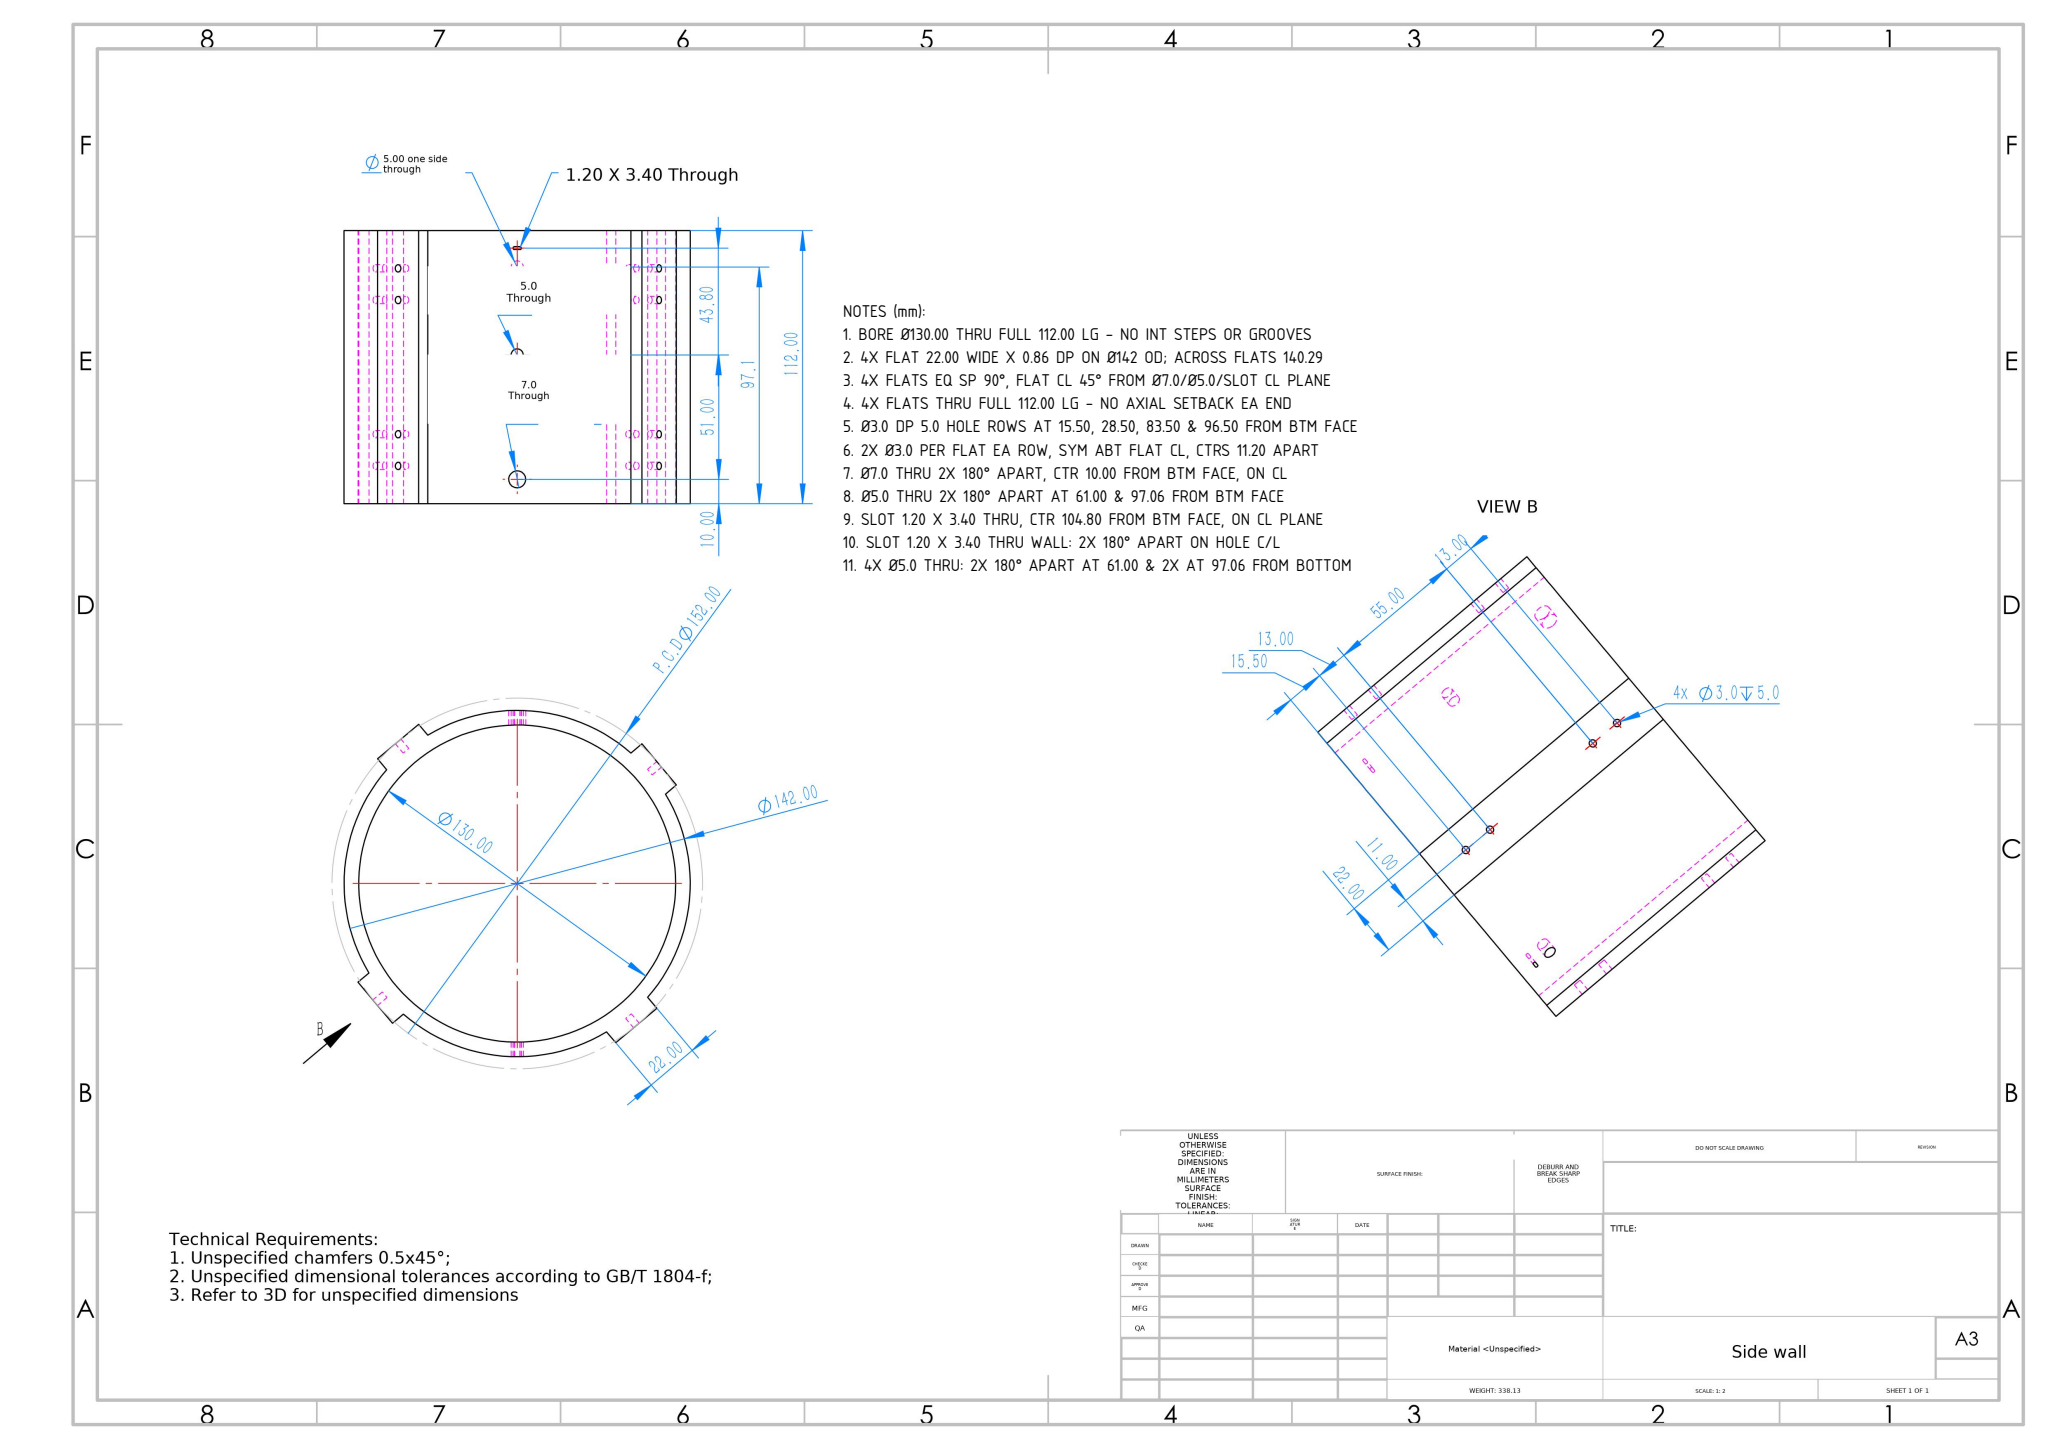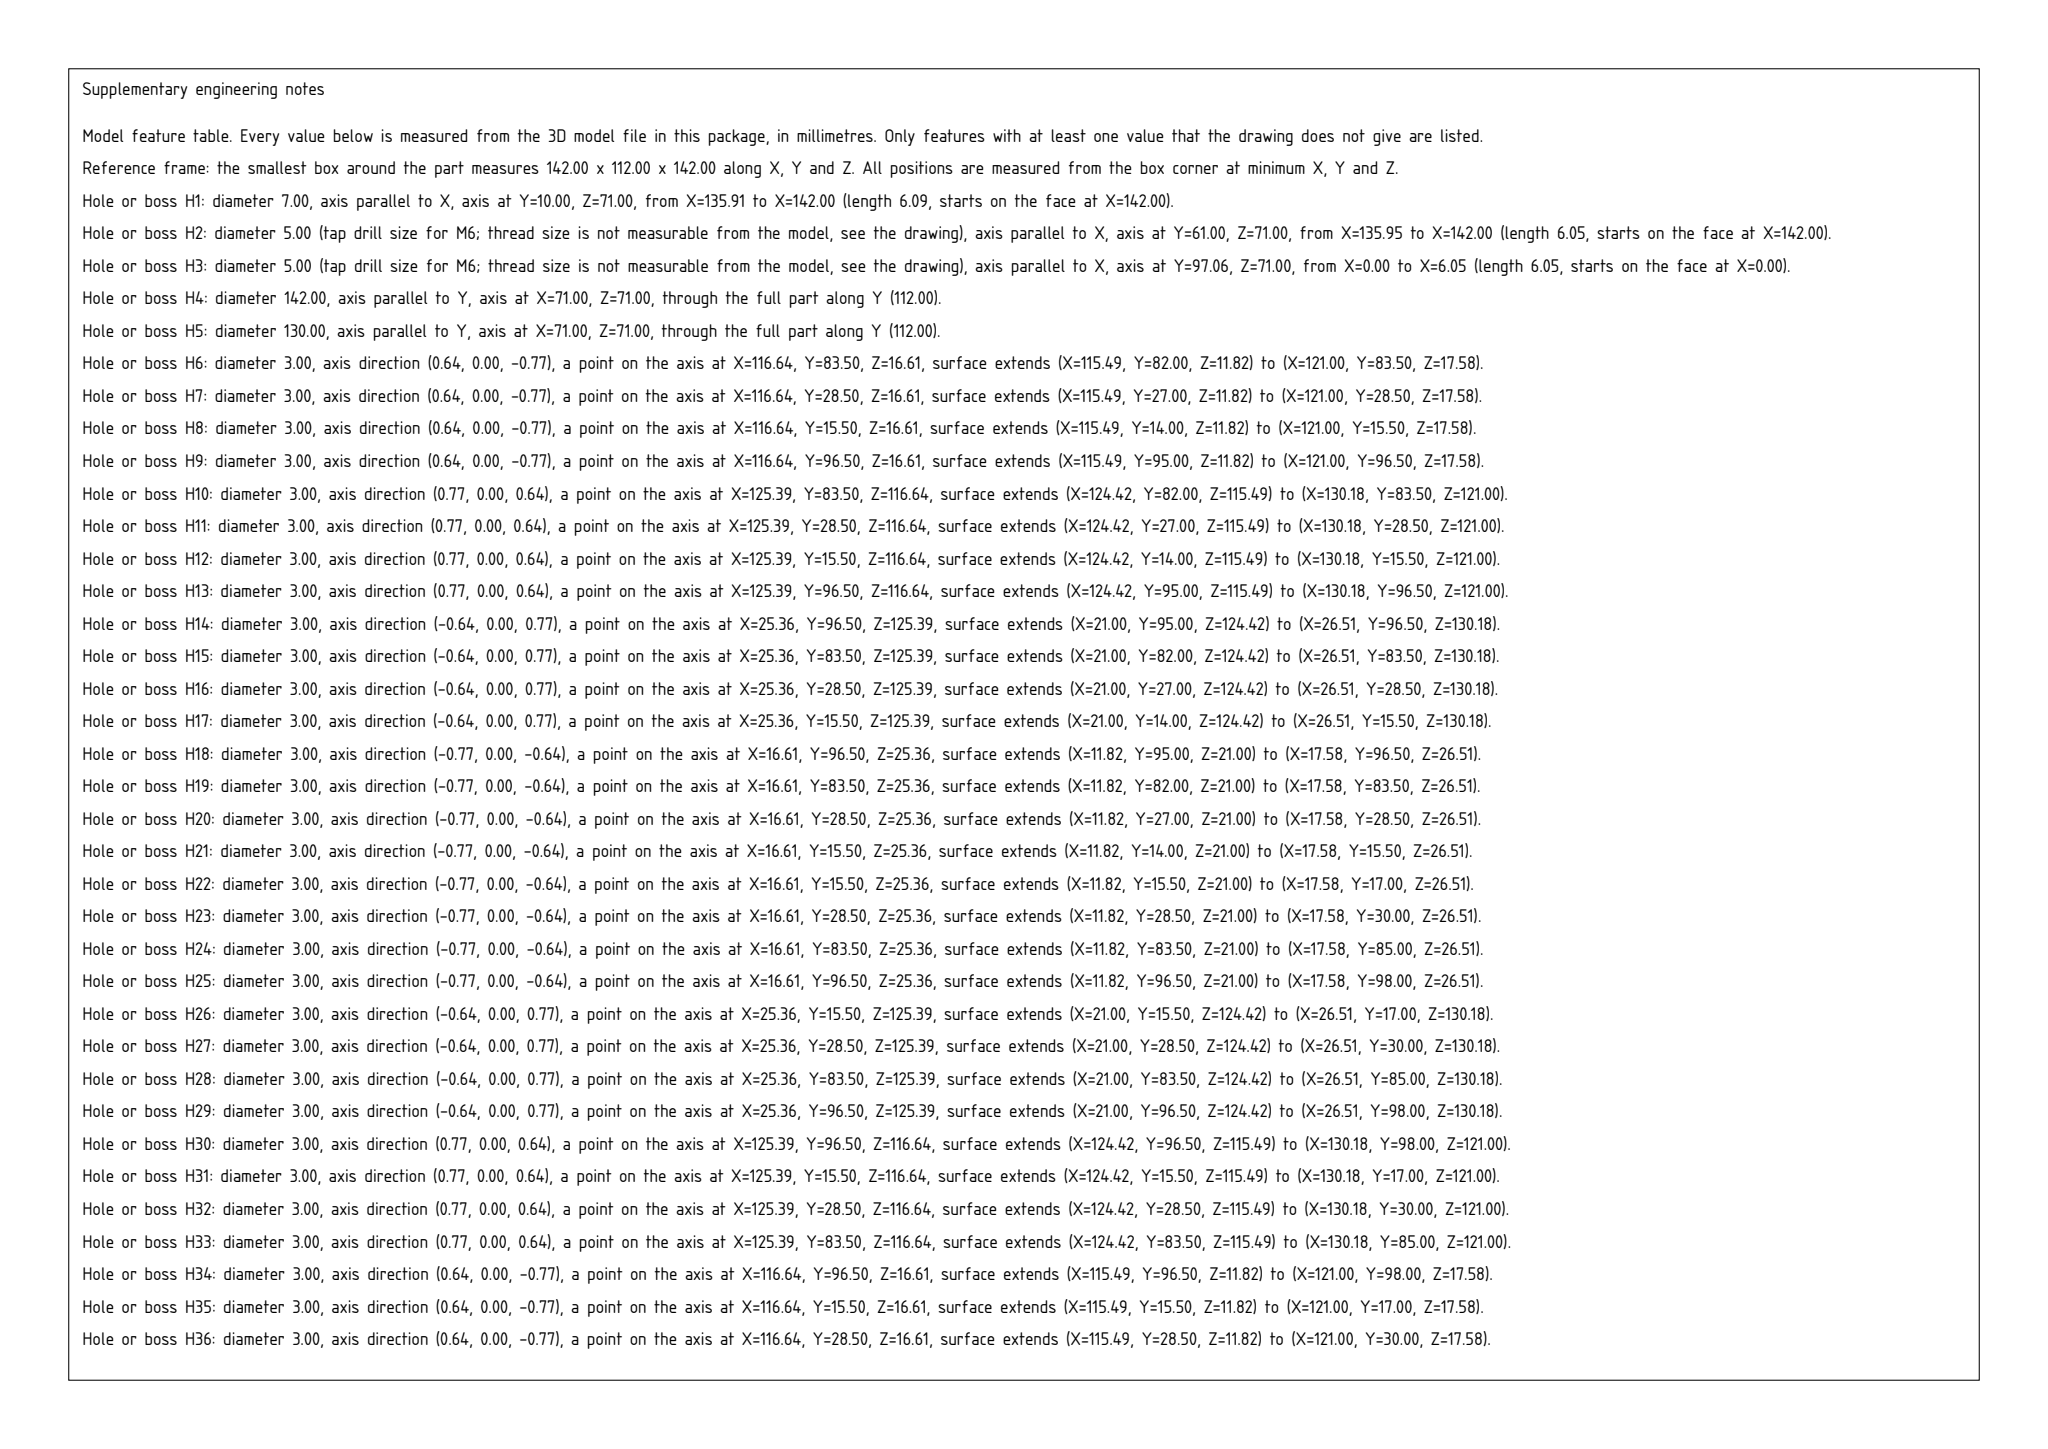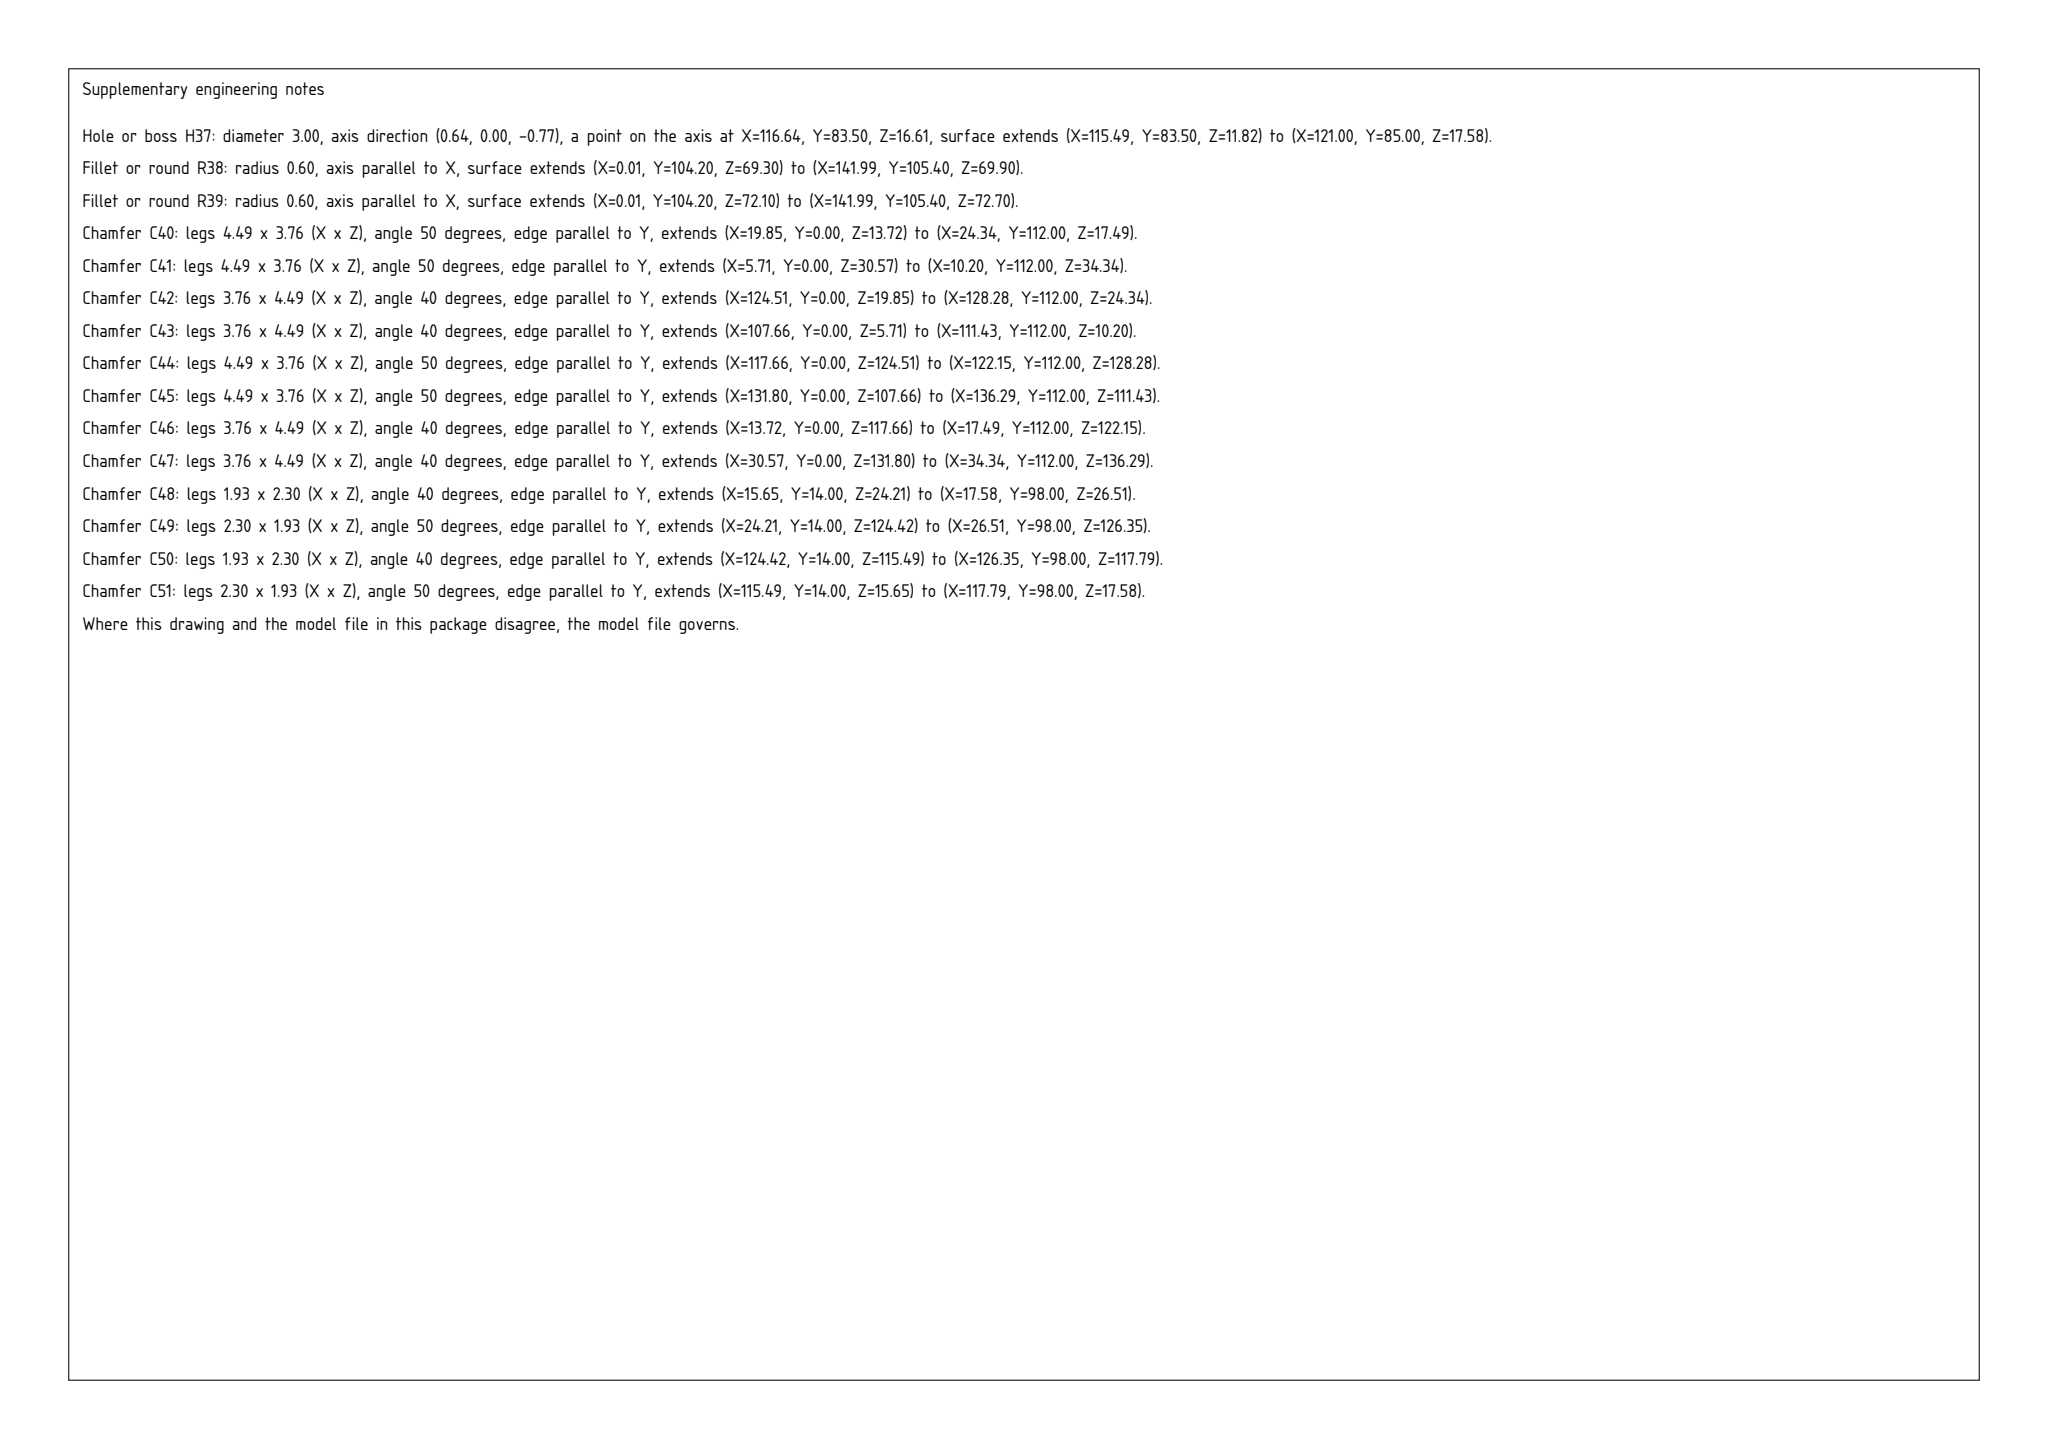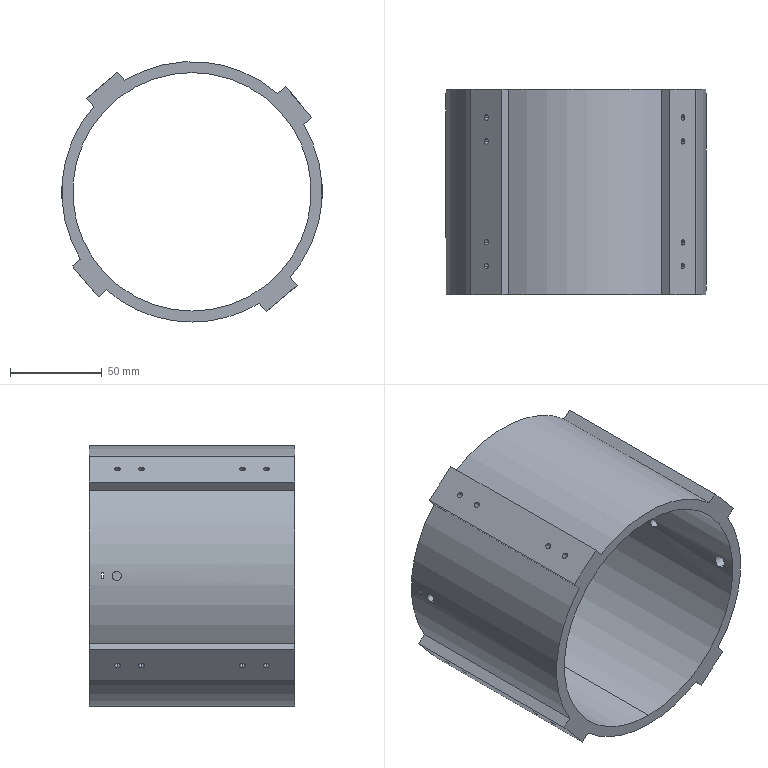Part | SolidWorks | mm | 1 solid | 85 faces | box 142 x 112 x 142 mm | volume 338129 mm3 | cylinder 51 | plane 34 | commonest cylinder face diameters 3 x32 1.2 x6 142 x5 5 x4 7 x2 130 x2
Drawing notes:
BORE Ø130.00 THRU FULL 112.00 LG - NO INT STEPS OR GROOVES | from the solid: Only cyls Ø130 and Ø142, axis y, length 112 full; no other bore faces
4X FLAT 22.00 WIDE X 0.86 DP ON Ø142 OD; ACROSS FLATS 140.29 | from the solid: Ø142 OD split into 5 cyl faces by 4 flats; chord 22 on R71 -> dp 0.857, A/F 140.285
4X FLATS EQ SP 90°, FLAT CL 45° FROM Ø7.0/Ø5.0/SLOT CL PLANE | from the solid: Ø7.0, Ø5.0 & 1.2x3.4 slot on z=71 CL; flat hole pairs centred on the 4 diagonals
4X FLATS THRU FULL 112.00 LG - NO AXIAL SETBACK EA END | from the solid: Ø142 cyl faces each 112.00 long (count 5), bbox y=112.0; flats run end face to end face
Ø3.0 DP 5.0 HOLE ROWS AT 15.50, 28.50, 83.50 & 96.50 FROM BTM FACE | from the solid: Ø3.0 x 5.76 deep cyls at y=15.5, 28.5, 83.5, 96.5 (5.0 flat DP), part 112 lg
2X Ø3.0 PER FLAT EA ROW, SYM ABT FLAT CL, CTRS 11.20 APART | from the solid: Ø3.0 axes at x/z=25.36 & 116.64; pair ctr dist sqrt(7.92²+7.92²)=11.20 on each flat
Ø7.0 THRU 2X 180° APART, CTR 10.00 FROM BTM FACE, ON CL | from the solid: [7.0,'x',[null,10.0,71.0],6.09,2] - z=71 = part CL, y=10 from min face
Ø5.0 THRU 2X 180° APART AT 61.00 & 97.06 FROM BTM FACE | from the solid: [5.0,'x',[null,61.0,71.0],6.05,2] and [5.0,'x',[null,97.06,71.0],6.05,2]
SLOT 1.20 X 3.40 THRU, CTR 104.80 FROM BTM FACE, ON CL PLANE | from the solid: Ø1.2 cyls, axis x, y=104.8, z=69.9 & 72.1 (3.4 overall); planes y=104.2/105.4
SLOT 1.20 X 3.40 THRU WALL: 2X 180° APART ON HOLE C/L | from the solid: dia-1.2 slot-end cyls at y=104.8, z=69.9 & 72.1, axis X, len 6.01 (=wall thk); only 2 wall crossings exist on that X line (x=0-6.01 and 135.99-142), i.e. 2 slots 180° apart on z=71 c/l
4X Ø5.0 THRU: 2X 180° APART AT 61.00 & 2X AT 97.06 FROM BOTTOM | from the solid: dia-5.0 cyls axis X, len 6.05: [y=61.0,z=71.0] count 2 and [y=97.06,z=71.0] count 2; z=71 = part c/l, so each pair is 180° apart; bottom face = plane y=0 (same datum as 10.00 to Ø7.0)